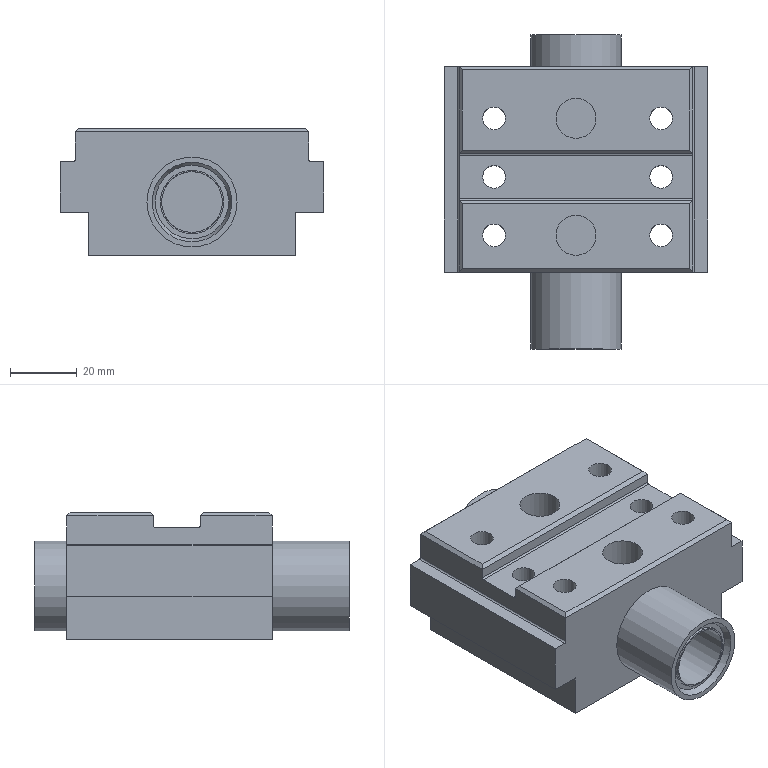Component | NX | MOVING_SLIDER_OTHER_HALF | 1 solid | 52 faces | volume 144746 mm3 | plane 34 | cylinder 17 | cone 1 | commonest cylinder face diameters 6.8 x6 1 x4 12 x2 27 x2 20 x1 19 x1 18.2 x1